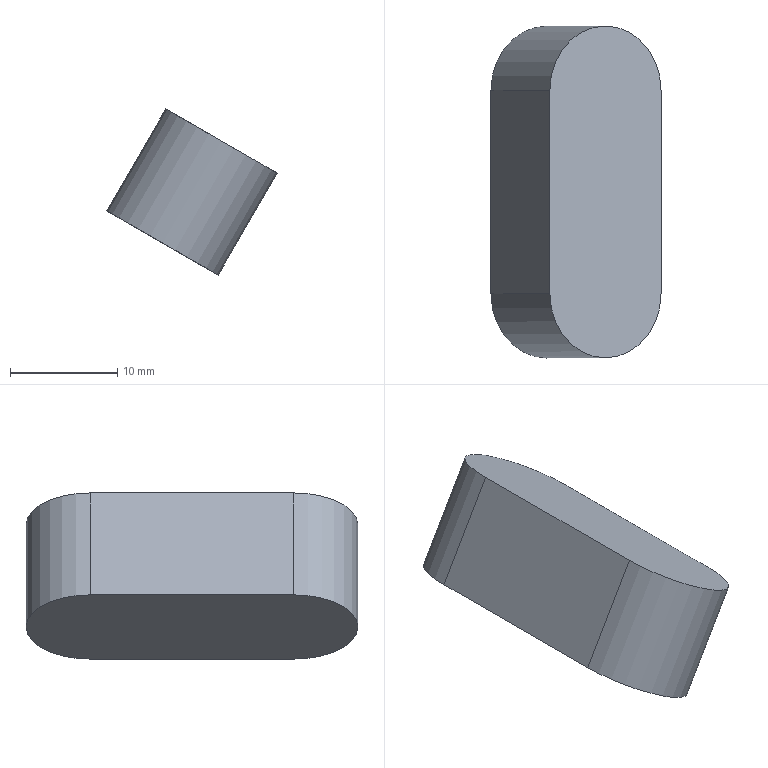Component | NX | KAMA | 1 solid | 6 faces | box 15.89 x 31 x 15.53 mm | volume 3752 mm3 | plane 4 | cylinder 2 | commonest cylinder face diameters 12 x2
STEP:
#1=CARTESIAN_POINT('',(0.,0.,0.));
#2=DIRECTION('',(0.,0.,1.));
#3=DIRECTION('',(1.,0.,0.));
#4=AXIS2_PLACEMENT_3D('',#1,#2,#3);
#5=CARTESIAN_POINT('',(-1151.062,819.425,240.321));
#6=VERTEX_POINT('',#5);
#7=CARTESIAN_POINT('',(-1140.67,819.425,234.321));
#8=VERTEX_POINT('',#7);
#9=CARTESIAN_POINT('',(-1145.866,819.425,237.321));
#10=DIRECTION('',(-0.5,0.,-0.866));
#11=DIRECTION('',(0.,-1.,0.));
#12=AXIS2_PLACEMENT_3D('',#9,#10,#11);
#13=CIRCLE('',#12,6.);
#14=CARTESIAN_POINT('',(-1140.366,819.425,246.847));
#15=DIRECTION('',(-0.5,0.,-0.866));
#16=DIRECTION('',(0.866,0.,-0.5));
#17=AXIS2_PLACEMENT_3D('',#14,#15,#16);
#18=CYLINDRICAL_SURFACE('',#17,6.);
#19=CARTESIAN_POINT('',(1.571,11.));
#20=DIRECTION('',(1.,-0.));
#21=VECTOR('',#20,1.);
#22=LINE('',#19,#21);
#23=(GEOMETRIC_REPRESENTATION_CONTEXT(2)PARAMETRIC_REPRESENTATION_CONTEXT()REPRESENTATION_CONTEXT('',''));
#24=DEFINITIONAL_REPRESENTATION('',(#22),#23);
#25=PCURVE('',#18,#24);
#26=CARTESIAN_POINT('',(-1145.866,819.425,237.321));
#27=DIRECTION('',(-0.5,0.,-0.866));
#28=DIRECTION('',(0.866,0.,-0.5));
#29=AXIS2_PLACEMENT_3D('',#26,#27,#28);
#30=PLANE('',#29);
#31=CARTESIAN_POINT('',(0.,0.));
#32=DIRECTION('',(0.,1.));
#33=AXIS2_PLACEMENT_2D('',#31,#32);
#34=CIRCLE('',#33,6.);
#35=(GEOMETRIC_REPRESENTATION_CONTEXT(2)PARAMETRIC_REPRESENTATION_CONTEXT()REPRESENTATION_CONTEXT('',''));
#36=DEFINITIONAL_REPRESENTATION('',(#34),#35);
#37=PCURVE('',#30,#36);
#38=SURFACE_CURVE('',#13,(#25,#37),.PCURVE_S1.);
#39=EDGE_CURVE('',#6,#8,#38,.T.);
#40=ORIENTED_EDGE('',*,*,#39,.F.);
#41=CARTESIAN_POINT('',(-1145.562,819.425,249.847));
#42=VERTEX_POINT('',#41);
#43=CARTESIAN_POINT('',(-1145.562,819.425,249.847));
#44=DIRECTION('',(-0.5,0.,-0.866));
#45=VECTOR('',#44,1.);
#46=LINE('',#43,#45);
#47=CARTESIAN_POINT('',(3.142,-0.));
#48=DIRECTION('',(0.,1.));
#49=VECTOR('',#48,1.);
#50=LINE('',#47,#49);
#51=(GEOMETRIC_REPRESENTATION_CONTEXT(2)PARAMETRIC_REPRESENTATION_CONTEXT()REPRESENTATION_CONTEXT('',''));
#52=DEFINITIONAL_REPRESENTATION('',(#50),#51);
#53=PCURVE('',#18,#52);
#54=CARTESIAN_POINT('',(-1145.562,800.425,249.847));
#55=DIRECTION('',(-0.866,0.,0.5));
#56=DIRECTION('',(-0.,-1.,0.));
#57=AXIS2_PLACEMENT_3D('',#54,#55,#56);
#58=PLANE('',#57);
#59=CARTESIAN_POINT('',(-19.,-0.));
#60=DIRECTION('',(0.,-1.));
#61=VECTOR('',#60,1.);
#62=LINE('',#59,#61);
#63=(GEOMETRIC_REPRESENTATION_CONTEXT(2)PARAMETRIC_REPRESENTATION_CONTEXT()REPRESENTATION_CONTEXT('',''));
#64=DEFINITIONAL_REPRESENTATION('',(#62),#63);
#65=PCURVE('',#58,#64);
#66=SURFACE_CURVE('',#46,(#53,#65),.PCURVE_S1.);
#67=EDGE_CURVE('',#42,#6,#66,.T.);
#68=ORIENTED_EDGE('',*,*,#67,.F.);
#69=CARTESIAN_POINT('',(-1135.17,819.425,243.847));
#70=VERTEX_POINT('',#69);
#71=CARTESIAN_POINT('',(-1140.366,819.425,246.847));
#72=DIRECTION('',(-0.5,0.,-0.866));
#73=DIRECTION('',(0.,-1.,0.));
#74=AXIS2_PLACEMENT_3D('',#71,#72,#73);
#75=CIRCLE('',#74,6.);
#76=CARTESIAN_POINT('',(1.571,0.));
#77=DIRECTION('',(1.,-0.));
#78=VECTOR('',#77,1.);
#79=LINE('',#76,#78);
#80=(GEOMETRIC_REPRESENTATION_CONTEXT(2)PARAMETRIC_REPRESENTATION_CONTEXT()REPRESENTATION_CONTEXT('',''));
#81=DEFINITIONAL_REPRESENTATION('',(#79),#80);
#82=PCURVE('',#18,#81);
#83=CARTESIAN_POINT('',(-1140.366,819.425,246.847));
#84=DIRECTION('',(-0.5,0.,-0.866));
#85=DIRECTION('',(0.866,0.,-0.5));
#86=AXIS2_PLACEMENT_3D('',#83,#84,#85);
#87=PLANE('',#86);
#88=CARTESIAN_POINT('',(0.,0.));
#89=DIRECTION('',(0.,1.));
#90=AXIS2_PLACEMENT_2D('',#88,#89);
#91=CIRCLE('',#90,6.);
#92=(GEOMETRIC_REPRESENTATION_CONTEXT(2)PARAMETRIC_REPRESENTATION_CONTEXT()REPRESENTATION_CONTEXT('',''));
#93=DEFINITIONAL_REPRESENTATION('',(#91),#92);
#94=PCURVE('',#87,#93);
#95=SURFACE_CURVE('',#75,(#82,#94),.PCURVE_S1.);
#96=EDGE_CURVE('',#42,#70,#95,.T.);
#97=ORIENTED_EDGE('',*,*,#96,.T.);
#98=CARTESIAN_POINT('',(-1135.17,819.425,243.847));
#99=DIRECTION('',(-0.5,0.,-0.866));
#100=VECTOR('',#99,1.);
#101=LINE('',#98,#100);
#102=CARTESIAN_POINT('',(6.283,-0.));
#103=DIRECTION('',(0.,1.));
#104=VECTOR('',#103,1.);
#105=LINE('',#102,#104);
#106=(GEOMETRIC_REPRESENTATION_CONTEXT(2)PARAMETRIC_REPRESENTATION_CONTEXT()REPRESENTATION_CONTEXT('',''));
#107=DEFINITIONAL_REPRESENTATION('',(#105),#106);
#108=PCURVE('',#18,#107);
#109=CARTESIAN_POINT('',(-1135.17,819.425,243.847));
#110=DIRECTION('',(0.866,-0.,-0.5));
#111=DIRECTION('',(0.,1.,-0.));
#112=AXIS2_PLACEMENT_3D('',#109,#110,#111);
#113=PLANE('',#112);
#114=CARTESIAN_POINT('',(-0.,0.));
#115=DIRECTION('',(-0.,-1.));
#116=VECTOR('',#115,1.);
#117=LINE('',#114,#116);
#118=(GEOMETRIC_REPRESENTATION_CONTEXT(2)PARAMETRIC_REPRESENTATION_CONTEXT()REPRESENTATION_CONTEXT('',''));
#119=DEFINITIONAL_REPRESENTATION('',(#117),#118);
#120=PCURVE('',#113,#119);
#121=SURFACE_CURVE('',#101,(#108,#120),.PCURVE_S1.);
#122=EDGE_CURVE('',#70,#8,#121,.T.);
#123=ORIENTED_EDGE('',*,*,#122,.T.);
#124=EDGE_LOOP('',(#40,#68,#97,#123));
#125=FACE_BOUND('',#124,.T.);
#126=ADVANCED_FACE('',(#125),#18,.T.);
#127=CARTESIAN_POINT('',(-1140.67,800.425,234.321));
#128=VERTEX_POINT('',#127);
#129=CARTESIAN_POINT('',(-1140.67,819.425,234.321));
#130=DIRECTION('',(-0.,-1.,0.));
#131=VECTOR('',#130,1.);
#132=LINE('',#129,#131);
#133=CARTESIAN_POINT('',(-0.,-11.));
#134=DIRECTION('',(-1.,0.));
#135=VECTOR('',#134,1.);
#136=LINE('',#133,#135);
#137=(GEOMETRIC_REPRESENTATION_CONTEXT(2)PARAMETRIC_REPRESENTATION_CONTEXT()REPRESENTATION_CONTEXT('',''));
#138=DEFINITIONAL_REPRESENTATION('',(#136),#137);
#139=PCURVE('',#113,#138);
#140=CARTESIAN_POINT('',(6.,0.));
#141=DIRECTION('',(-0.,1.));
#142=VECTOR('',#141,1.);
#143=LINE('',#140,#142);
#144=(GEOMETRIC_REPRESENTATION_CONTEXT(2)PARAMETRIC_REPRESENTATION_CONTEXT()REPRESENTATION_CONTEXT('',''));
#145=DEFINITIONAL_REPRESENTATION('',(#143),#144);
#146=PCURVE('',#30,#145);
#147=SURFACE_CURVE('',#132,(#139,#146),.PCURVE_S1.);
#148=EDGE_CURVE('',#8,#128,#147,.T.);
#149=ORIENTED_EDGE('',*,*,#148,.F.);
#150=ORIENTED_EDGE('',*,*,#122,.F.);
#151=CARTESIAN_POINT('',(-1135.17,800.425,243.847));
#152=VERTEX_POINT('',#151);
#153=CARTESIAN_POINT('',(-1135.17,819.425,243.847));
#154=DIRECTION('',(-0.,-1.,0.));
#155=VECTOR('',#154,1.);
#156=LINE('',#153,#155);
#157=CARTESIAN_POINT('',(0.,0.));
#158=DIRECTION('',(-1.,0.));
#159=VECTOR('',#158,1.);
#160=LINE('',#157,#159);
#161=(GEOMETRIC_REPRESENTATION_CONTEXT(2)PARAMETRIC_REPRESENTATION_CONTEXT()REPRESENTATION_CONTEXT('',''));
#162=DEFINITIONAL_REPRESENTATION('',(#160),#161);
#163=PCURVE('',#113,#162);
#164=CARTESIAN_POINT('',(6.,0.));
#165=DIRECTION('',(-0.,1.));
#166=VECTOR('',#165,1.);
#167=LINE('',#164,#166);
#168=(GEOMETRIC_REPRESENTATION_CONTEXT(2)PARAMETRIC_REPRESENTATION_CONTEXT()REPRESENTATION_CONTEXT('',''));
#169=DEFINITIONAL_REPRESENTATION('',(#167),#168);
#170=PCURVE('',#87,#169);
#171=SURFACE_CURVE('',#156,(#163,#170),.PCURVE_S1.);
#172=EDGE_CURVE('',#70,#152,#171,.T.);
#173=ORIENTED_EDGE('',*,*,#172,.T.);
#174=CARTESIAN_POINT('',(-1135.17,800.425,243.847));
#175=DIRECTION('',(-0.5,0.,-0.866));
#176=VECTOR('',#175,1.);
#177=LINE('',#174,#176);
#178=CARTESIAN_POINT('',(-19.,0.));
#179=DIRECTION('',(-0.,-1.));
#180=VECTOR('',#179,1.);
#181=LINE('',#178,#180);
#182=(GEOMETRIC_REPRESENTATION_CONTEXT(2)PARAMETRIC_REPRESENTATION_CONTEXT()REPRESENTATION_CONTEXT('',''));
#183=DEFINITIONAL_REPRESENTATION('',(#181),#182);
#184=PCURVE('',#113,#183);
#185=CARTESIAN_POINT('',(-1140.366,800.425,246.847));
#186=DIRECTION('',(-0.5,0.,-0.866));
#187=DIRECTION('',(0.866,0.,-0.5));
#188=AXIS2_PLACEMENT_3D('',#185,#186,#187);
#189=CYLINDRICAL_SURFACE('',#188,6.);
#190=CARTESIAN_POINT('',(0.,-0.));
#191=DIRECTION('',(0.,1.));
#192=VECTOR('',#191,1.);
#193=LINE('',#190,#192);
#194=(GEOMETRIC_REPRESENTATION_CONTEXT(2)PARAMETRIC_REPRESENTATION_CONTEXT()REPRESENTATION_CONTEXT('',''));
#195=DEFINITIONAL_REPRESENTATION('',(#193),#194);
#196=PCURVE('',#189,#195);
#197=SURFACE_CURVE('',#177,(#184,#196),.PCURVE_S1.);
#198=EDGE_CURVE('',#152,#128,#197,.T.);
#199=ORIENTED_EDGE('',*,*,#198,.T.);
#200=EDGE_LOOP('',(#149,#150,#173,#199));
#201=FACE_BOUND('',#200,.T.);
#202=ADVANCED_FACE('',(#201),#113,.T.);
#203=CARTESIAN_POINT('',(-1151.062,800.425,240.321));
#204=VERTEX_POINT('',#203);
#205=CARTESIAN_POINT('',(-1145.866,800.425,237.321));
#206=DIRECTION('',(-0.5,0.,-0.866));
#207=DIRECTION('',(0.,1.,0.));
#208=AXIS2_PLACEMENT_3D('',#205,#206,#207);
#209=CIRCLE('',#208,6.);
#210=CARTESIAN_POINT('',(-1.571,11.));
#211=DIRECTION('',(1.,0.));
#212=VECTOR('',#211,1.);
#213=LINE('',#210,#212);
#214=(GEOMETRIC_REPRESENTATION_CONTEXT(2)PARAMETRIC_REPRESENTATION_CONTEXT()REPRESENTATION_CONTEXT('',''));
#215=DEFINITIONAL_REPRESENTATION('',(#213),#214);
#216=PCURVE('',#189,#215);
#217=CARTESIAN_POINT('',(0.,19.));
#218=DIRECTION('',(0.,-1.));
#219=AXIS2_PLACEMENT_2D('',#217,#218);
#220=CIRCLE('',#219,6.);
#221=(GEOMETRIC_REPRESENTATION_CONTEXT(2)PARAMETRIC_REPRESENTATION_CONTEXT()REPRESENTATION_CONTEXT('',''));
#222=DEFINITIONAL_REPRESENTATION('',(#220),#221);
#223=PCURVE('',#30,#222);
#224=SURFACE_CURVE('',#209,(#216,#223),.PCURVE_S1.);
#225=EDGE_CURVE('',#128,#204,#224,.T.);
#226=ORIENTED_EDGE('',*,*,#225,.F.);
#227=ORIENTED_EDGE('',*,*,#198,.F.);
#228=CARTESIAN_POINT('',(-1145.562,800.425,249.847));
#229=VERTEX_POINT('',#228);
#230=CARTESIAN_POINT('',(-1140.366,800.425,246.847));
#231=DIRECTION('',(-0.5,0.,-0.866));
#232=DIRECTION('',(0.,1.,0.));
#233=AXIS2_PLACEMENT_3D('',#230,#231,#232);
#234=CIRCLE('',#233,6.);
#235=CARTESIAN_POINT('',(-1.571,-0.));
#236=DIRECTION('',(1.,0.));
#237=VECTOR('',#236,1.);
#238=LINE('',#235,#237);
#239=(GEOMETRIC_REPRESENTATION_CONTEXT(2)PARAMETRIC_REPRESENTATION_CONTEXT()REPRESENTATION_CONTEXT('',''));
#240=DEFINITIONAL_REPRESENTATION('',(#238),#239);
#241=PCURVE('',#189,#240);
#242=CARTESIAN_POINT('',(0.,19.));
#243=DIRECTION('',(0.,-1.));
#244=AXIS2_PLACEMENT_2D('',#242,#243);
#245=CIRCLE('',#244,6.);
#246=(GEOMETRIC_REPRESENTATION_CONTEXT(2)PARAMETRIC_REPRESENTATION_CONTEXT()REPRESENTATION_CONTEXT('',''));
#247=DEFINITIONAL_REPRESENTATION('',(#245),#246);
#248=PCURVE('',#87,#247);
#249=SURFACE_CURVE('',#234,(#241,#248),.PCURVE_S1.);
#250=EDGE_CURVE('',#152,#229,#249,.T.);
#251=ORIENTED_EDGE('',*,*,#250,.T.);
#252=CARTESIAN_POINT('',(-1145.562,800.425,249.847));
#253=DIRECTION('',(-0.5,0.,-0.866));
#254=VECTOR('',#253,1.);
#255=LINE('',#252,#254);
#256=CARTESIAN_POINT('',(3.142,-0.));
#257=DIRECTION('',(0.,1.));
#258=VECTOR('',#257,1.);
#259=LINE('',#256,#258);
#260=(GEOMETRIC_REPRESENTATION_CONTEXT(2)PARAMETRIC_REPRESENTATION_CONTEXT()REPRESENTATION_CONTEXT('',''));
#261=DEFINITIONAL_REPRESENTATION('',(#259),#260);
#262=PCURVE('',#189,#261);
#263=CARTESIAN_POINT('',(-0.,-0.));
#264=DIRECTION('',(0.,-1.));
#265=VECTOR('',#264,1.);
#266=LINE('',#263,#265);
#267=(GEOMETRIC_REPRESENTATION_CONTEXT(2)PARAMETRIC_REPRESENTATION_CONTEXT()REPRESENTATION_CONTEXT('',''));
#268=DEFINITIONAL_REPRESENTATION('',(#266),#267);
#269=PCURVE('',#58,#268);
#270=SURFACE_CURVE('',#255,(#262,#269),.PCURVE_S1.);
#271=EDGE_CURVE('',#229,#204,#270,.T.);
#272=ORIENTED_EDGE('',*,*,#271,.T.);
#273=EDGE_LOOP('',(#226,#227,#251,#272));
#274=FACE_BOUND('',#273,.T.);
#275=ADVANCED_FACE('',(#274),#189,.T.);
#276=CARTESIAN_POINT('',(-1151.062,800.425,240.321));
#277=DIRECTION('',(0.,1.,-0.));
#278=VECTOR('',#277,1.);
#279=LINE('',#276,#278);
#280=CARTESIAN_POINT('',(0.,-11.));
#281=DIRECTION('',(-1.,-0.));
#282=VECTOR('',#281,1.);
#283=LINE('',#280,#282);
#284=(GEOMETRIC_REPRESENTATION_CONTEXT(2)PARAMETRIC_REPRESENTATION_CONTEXT()REPRESENTATION_CONTEXT('',''));
#285=DEFINITIONAL_REPRESENTATION('',(#283),#284);
#286=PCURVE('',#58,#285);
#287=CARTESIAN_POINT('',(-6.,19.));
#288=DIRECTION('',(0.,-1.));
#289=VECTOR('',#288,1.);
#290=LINE('',#287,#289);
#291=(GEOMETRIC_REPRESENTATION_CONTEXT(2)PARAMETRIC_REPRESENTATION_CONTEXT()REPRESENTATION_CONTEXT('',''));
#292=DEFINITIONAL_REPRESENTATION('',(#290),#291);
#293=PCURVE('',#30,#292);
#294=SURFACE_CURVE('',#279,(#286,#293),.PCURVE_S1.);
#295=EDGE_CURVE('',#204,#6,#294,.T.);
#296=ORIENTED_EDGE('',*,*,#295,.F.);
#297=ORIENTED_EDGE('',*,*,#271,.F.);
#298=CARTESIAN_POINT('',(-1145.562,800.425,249.847));
#299=DIRECTION('',(0.,1.,-0.));
#300=VECTOR('',#299,1.);
#301=LINE('',#298,#300);
#302=CARTESIAN_POINT('',(0.,0.));
#303=DIRECTION('',(-1.,-0.));
#304=VECTOR('',#303,1.);
#305=LINE('',#302,#304);
#306=(GEOMETRIC_REPRESENTATION_CONTEXT(2)PARAMETRIC_REPRESENTATION_CONTEXT()REPRESENTATION_CONTEXT('',''));
#307=DEFINITIONAL_REPRESENTATION('',(#305),#306);
#308=PCURVE('',#58,#307);
#309=CARTESIAN_POINT('',(-6.,19.));
#310=DIRECTION('',(0.,-1.));
#311=VECTOR('',#310,1.);
#312=LINE('',#309,#311);
#313=(GEOMETRIC_REPRESENTATION_CONTEXT(2)PARAMETRIC_REPRESENTATION_CONTEXT()REPRESENTATION_CONTEXT('',''));
#314=DEFINITIONAL_REPRESENTATION('',(#312),#313);
#315=PCURVE('',#87,#314);
#316=SURFACE_CURVE('',#301,(#308,#315),.PCURVE_S1.);
#317=EDGE_CURVE('',#229,#42,#316,.T.);
#318=ORIENTED_EDGE('',*,*,#317,.T.);
#319=ORIENTED_EDGE('',*,*,#67,.T.);
#320=EDGE_LOOP('',(#296,#297,#318,#319));
#321=FACE_BOUND('',#320,.T.);
#322=ADVANCED_FACE('',(#321),#58,.T.);
#323=ORIENTED_EDGE('',*,*,#96,.F.);
#324=ORIENTED_EDGE('',*,*,#317,.F.);
#325=ORIENTED_EDGE('',*,*,#250,.F.);
#326=ORIENTED_EDGE('',*,*,#172,.F.);
#327=EDGE_LOOP('',(#323,#324,#325,#326));
#328=FACE_BOUND('',#327,.T.);
#329=ADVANCED_FACE('',(#328),#87,.F.);
#330=ORIENTED_EDGE('',*,*,#39,.T.);
#331=ORIENTED_EDGE('',*,*,#148,.T.);
#332=ORIENTED_EDGE('',*,*,#225,.T.);
#333=ORIENTED_EDGE('',*,*,#295,.T.);
#334=EDGE_LOOP('',(#330,#331,#332,#333));
#335=FACE_BOUND('',#334,.T.);
#336=ADVANCED_FACE('',(#335),#30,.T.);
#337=CLOSED_SHELL('',(#126,#202,#275,#322,#329,#336));
#338=MANIFOLD_SOLID_BREP('',#337);
#339=(LENGTH_UNIT()NAMED_UNIT(*)SI_UNIT(.MILLI.,.METRE.));
#340=UNCERTAINTY_MEASURE_WITH_UNIT(LENGTH_MEASURE(0.0000001),#339,'','');
#341=(NAMED_UNIT(*)PLANE_ANGLE_UNIT()SI_UNIT($,.RADIAN.));
#342=(NAMED_UNIT(*)SI_UNIT($,.STERADIAN.)SOLID_ANGLE_UNIT());
#343=(GEOMETRIC_REPRESENTATION_CONTEXT(3)GLOBAL_UNCERTAINTY_ASSIGNED_CONTEXT((#340))GLOBAL_UNIT_ASSIGNED_CONTEXT((#339,#341,#342))REPRESENTATION_CONTEXT('',''));
#344=ADVANCED_BREP_SHAPE_REPRESENTATION('',(#4,#338),#343);